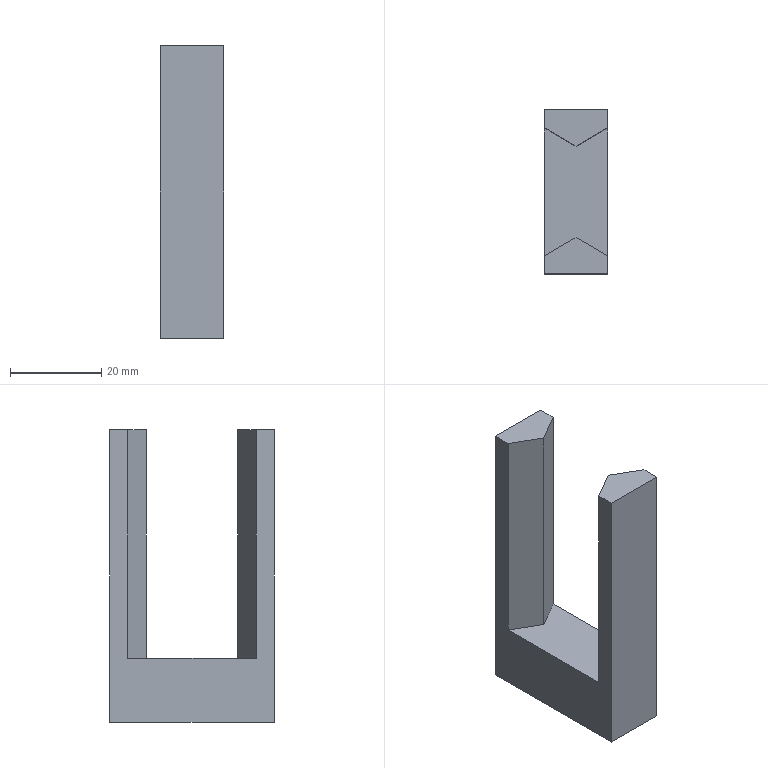Component | NX | 6_FORK | 1 solid | 18 faces | volume 14770 mm3 | plane 12 | cone 3 | cylinder 3 | commonest cylinder face diameters 4 x2 4.2 x1